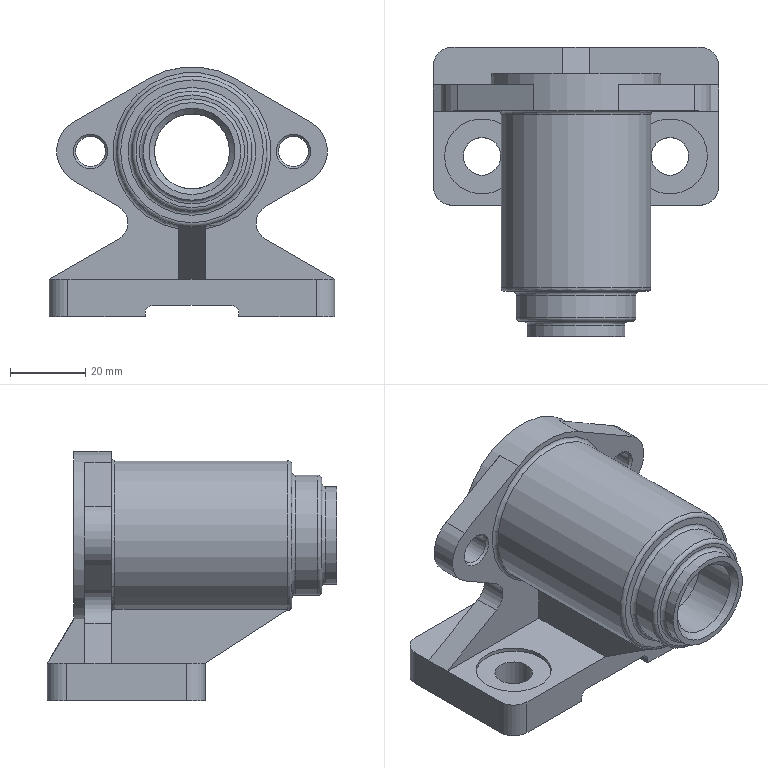Component | NX | PUMP_BODY | 1 solid | 72 faces | volume 82386 mm3 | plane 38 | cylinder 24 | cone 5 | torus 5 | commonest cylinder face diameters 10 x8 20 x3 40 x2 18 x2 32 x2 8 x2 4 x2 45 x1